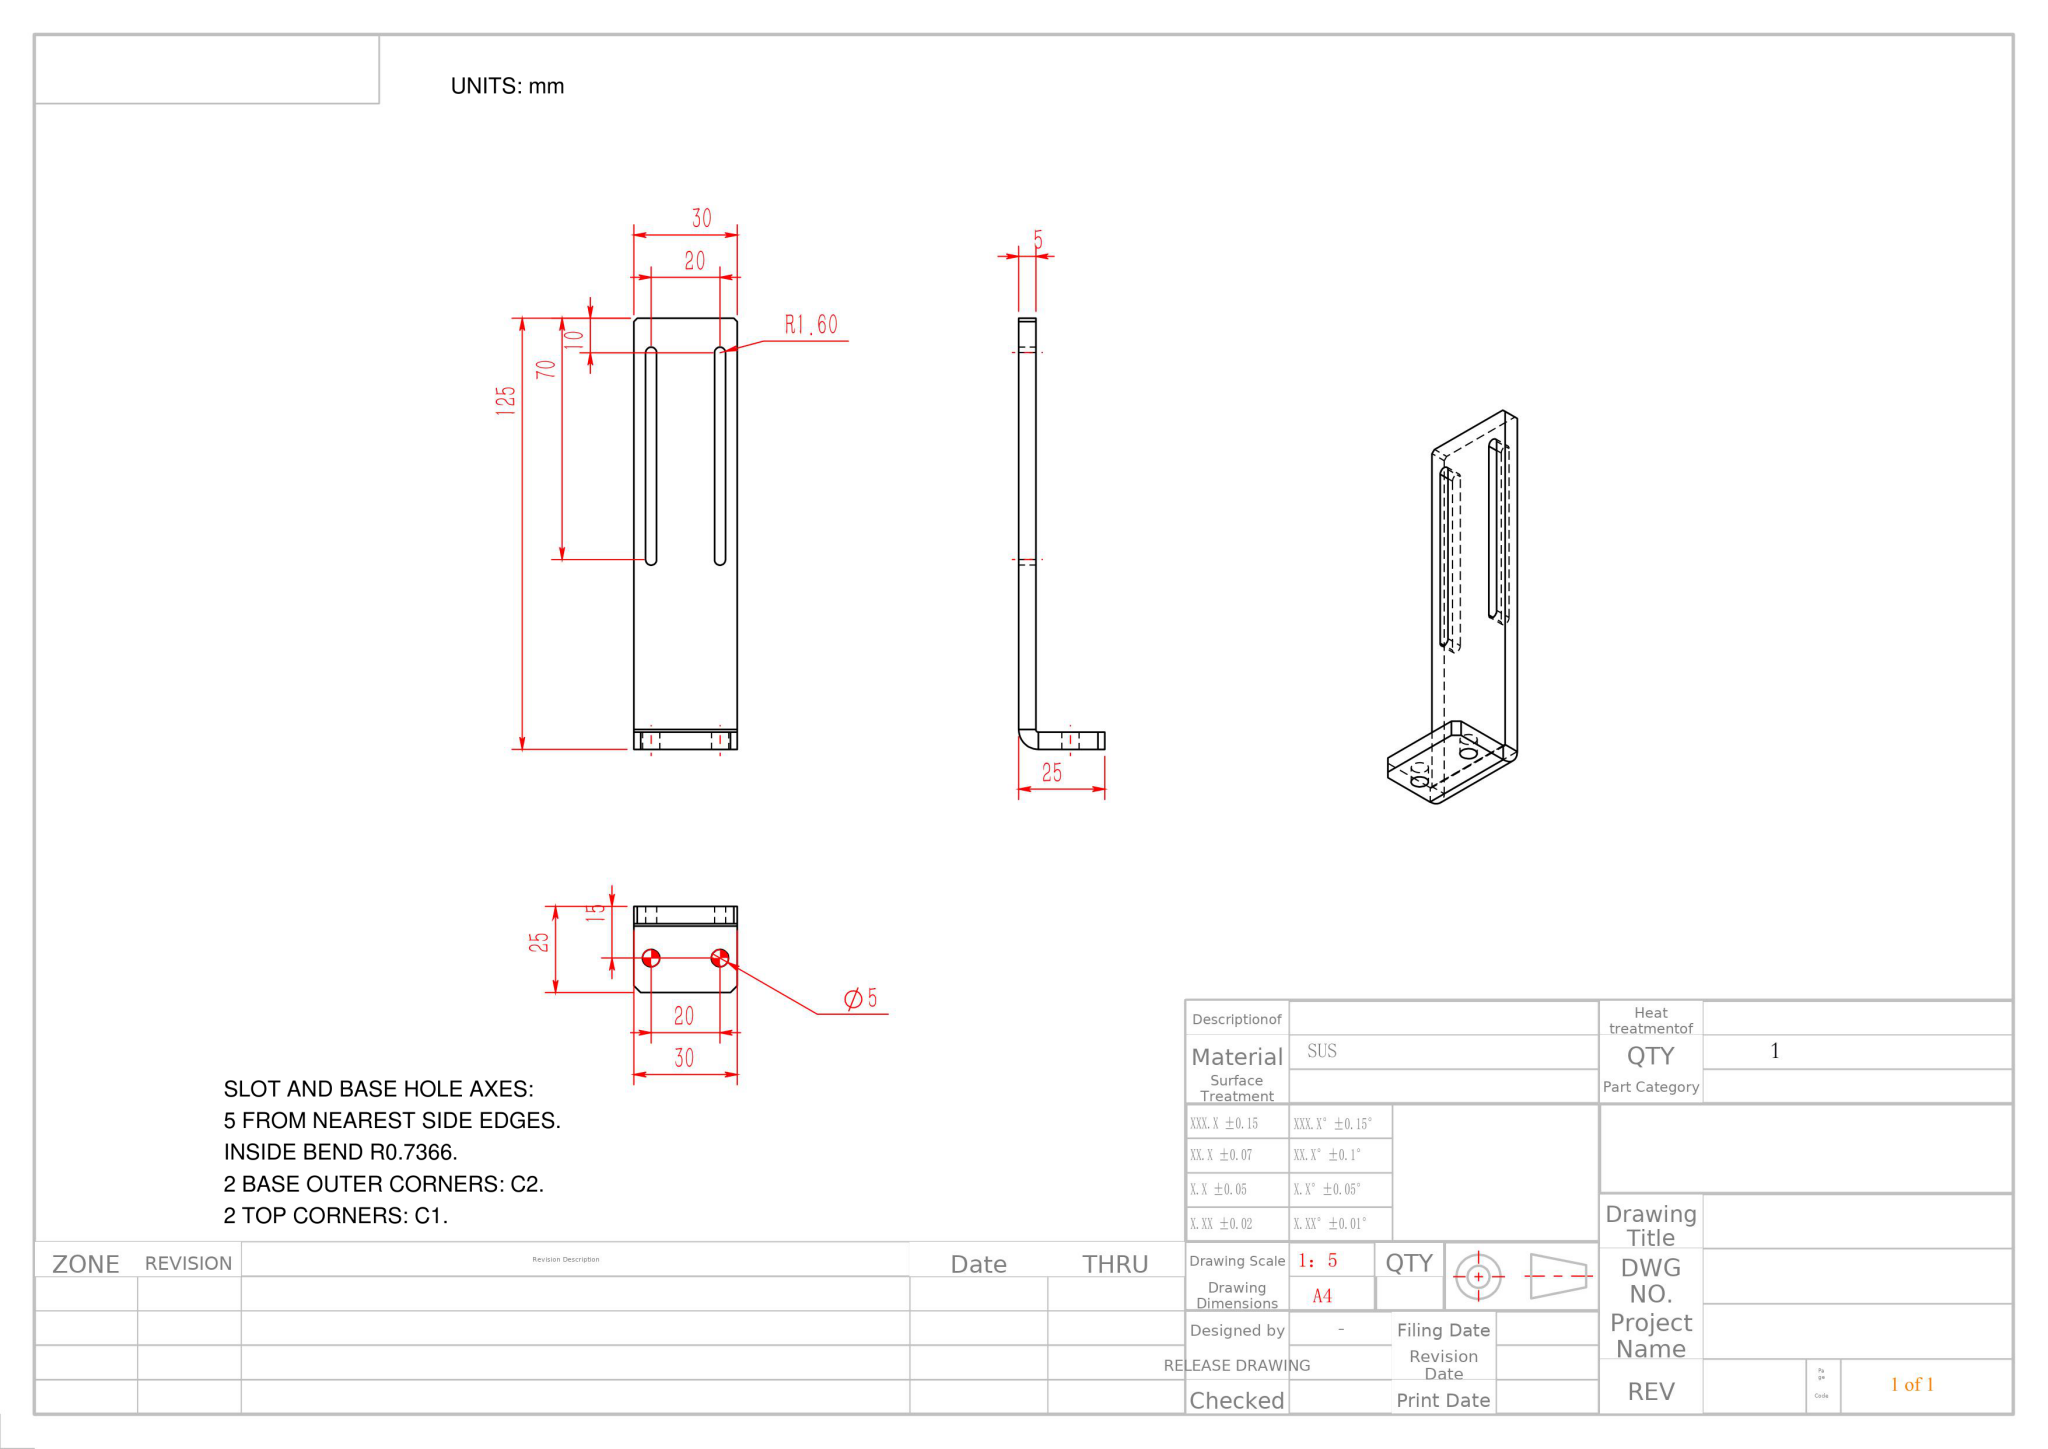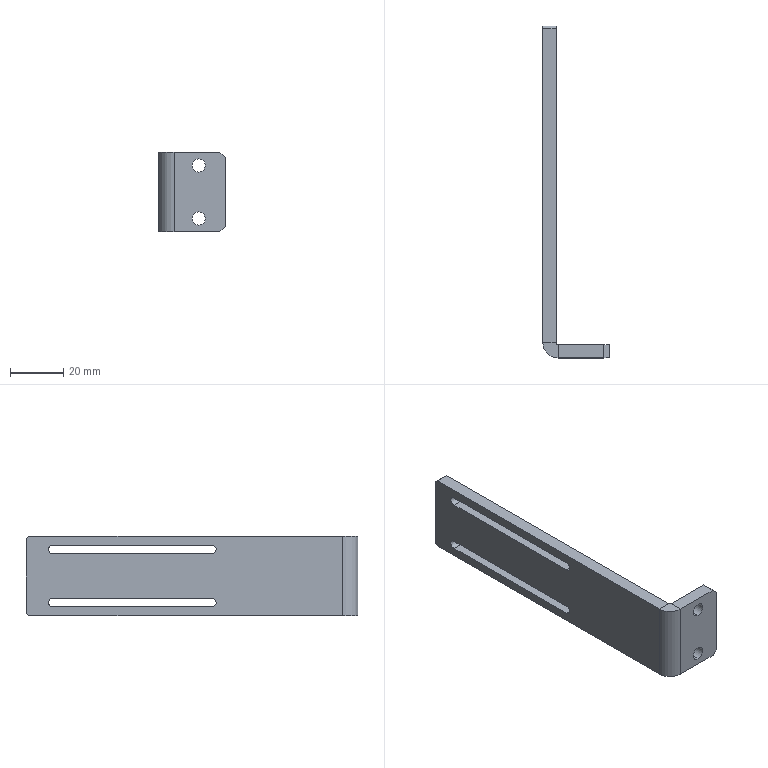Part | NX | mm | 1 solid | 30 faces | box 25 x 125 x 30 mm | volume 19320 mm3 | plane 20 | cylinder 10 | commonest cylinder face diameters 5 x4 3.2 x4 1.473 x1 11.473 x1